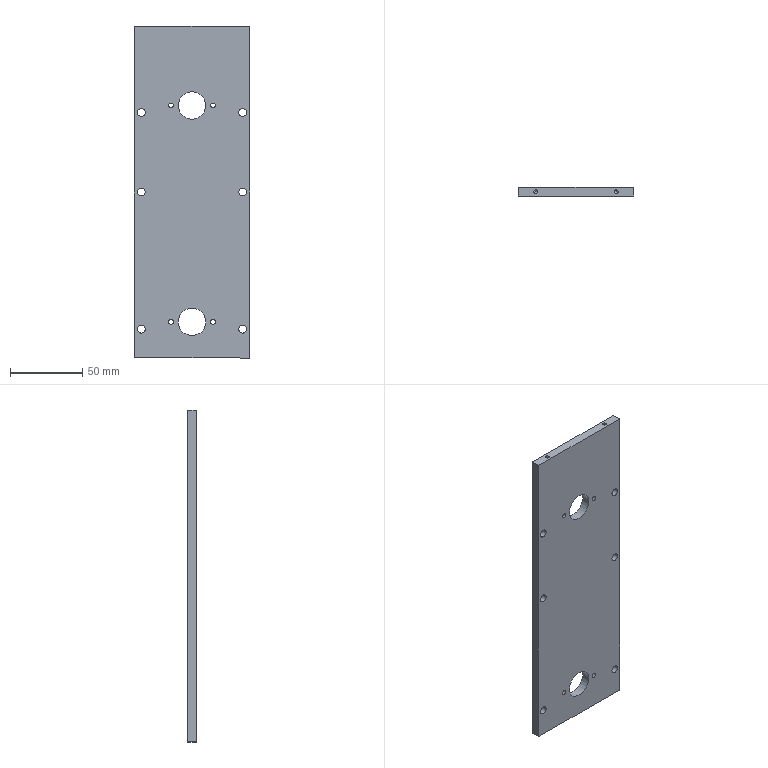Component | SolidWorks | 008-2 | 1 solid | 42 faces | box 80 x 6 x 230 mm | volume 105858 mm3 | cylinder 28 | plane 10 | cone 4 | commonest cylinder face diameters 5.5 x12 3.3 x8 2.5 x4 19 x4 | material AL6061
build123d program:
from build123d import *

# Parameters (mm, degrees)
SKETCH1_W                  = 80
SKETCH1_H                  = 240
BOSS_EXTRUDE1_DEPTH        = 6
SKETCH4_R                  = 2.75
CUT_EXTRUDE1_DEPTH         = 127.633
CHAMFER1_SIZE              = 0.5
SKETCH10_R                 = 9.5
CUT_EXTRUDE5_DEPTH         = 127.633
M4_TAPPED_HOLE2_D          = 3.3
M4_TAPPED_HOLE2_DEPTH      = 10.1
M4_TAPPED_HOLE2_TIP        = 0.9914
SKETCH19_W                 = 114.639
SKETCH19_H                 = 27.657
CUT_EXTRUDE7_DEPTH         = 127.633
CHAMFER2_SIZE              = 0.5
F_5_5_5_5_DIAMETER_HOLE1_D = 5.5
M3_TAPPED_HOLE2_D          = 2.5
M3_TAPPED_HOLE2_DEPTH      = 7.5
M3_TAPPED_HOLE2_TIP        = 0.7511


with BuildPart() as part:
    # Sketch1 → Boss-Extrude1 (new body)
    with BuildSketch(Plane.XY):
        Rectangle(SKETCH1_W, SKETCH1_H)
    extrude(amount=BOSS_EXTRUDE1_DEPTH)

    # Sketch4 → Cut-Extrude1 (cut, through all)
    with BuildSketch(Plane(origin=(0, 0, 0), x_dir=(-1, 0, 0), z_dir=(0, 0, -1))):
        with Locations((0, 115)):
            Circle(SKETCH4_R)
        with Locations((38, 115)):
            Circle(SKETCH4_R)
        with Locations((-38, 115)):
            Circle(SKETCH4_R)
    extrude(amount=-CUT_EXTRUDE1_DEPTH, mode=Mode.SUBTRACT)

    # Chamfer1
    chamfer1_edges = [part.edges().sort_by_distance(p)[0] for p in [
        (40, -120, 3),
        (-40, -120, 3),
        (-40, 120, 3),
        (40, 120, 3),
    ]]
    chamfer(chamfer1_edges, length=CHAMFER1_SIZE)

    # Sketch10 → Cut-Extrude5 (cut, through all)
    with BuildSketch(Plane.XY.offset(6)):
        with Locations((0, -95)):
            Circle(SKETCH10_R)
        with Locations((0, 55)):
            Circle(SKETCH10_R)
    extrude(amount=-CUT_EXTRUDE5_DEPTH, mode=Mode.SUBTRACT)

    # M4 Tapped Hole2
    with Locations(Plane.XY.offset(6)):
        with Locations((-14.5, -95), (14.5, -95), (14.5, 55), (-14.5, 55)):
            Hole(M4_TAPPED_HOLE2_D / 2, depth=M4_TAPPED_HOLE2_DEPTH)
            with Locations((0, 0, -(M4_TAPPED_HOLE2_DEPTH + M4_TAPPED_HOLE2_TIP / 2))):  # 118° drill point
                Cone(0, M4_TAPPED_HOLE2_D / 2, M4_TAPPED_HOLE2_TIP, mode=Mode.SUBTRACT)

    # Sketch19 → Cut-Extrude7 (cut, through all)
    with BuildSketch(Plane.XY.offset(6)):
        with Locations((2.436, 123.828)):
            Rectangle(SKETCH19_W, SKETCH19_H)
    extrude(amount=-CUT_EXTRUDE7_DEPTH, mode=Mode.SUBTRACT)

    # Chamfer2
    chamfer2_edges = [part.edges().sort_by_distance(p)[0] for p in [
        (-40, 110, 3),
        (40, 110, 3),
    ]]
    chamfer(chamfer2_edges, length=CHAMFER2_SIZE)

    # 5.5 _5.5_ Diameter Hole1 (through all)
    with Locations(Plane.XY.offset(6)):
        with Locations((-35, -100), (-35, -5), (-35, 50), (35, -100), (35, -5), (35, 50)):
            Hole(F_5_5_5_5_DIAMETER_HOLE1_D / 2)

    # M3 Tapped Hole2
    with Locations(Plane(origin=(0, 110, 0), x_dir=(1, 0, 0), z_dir=(0, 1, 0))):
        with Locations((28, -3), (-28, -3)):
            Hole(M3_TAPPED_HOLE2_D / 2, depth=M3_TAPPED_HOLE2_DEPTH)
            with Locations((0, 0, -(M3_TAPPED_HOLE2_DEPTH + M3_TAPPED_HOLE2_TIP / 2))):  # 118° drill point
                Cone(0, M3_TAPPED_HOLE2_D / 2, M3_TAPPED_HOLE2_TIP, mode=Mode.SUBTRACT)


solid = part.part

# Placed as in the assembly
solid = solid.moved(Location((-240.455, -145.942, -238.376), (90, 0, 0)))